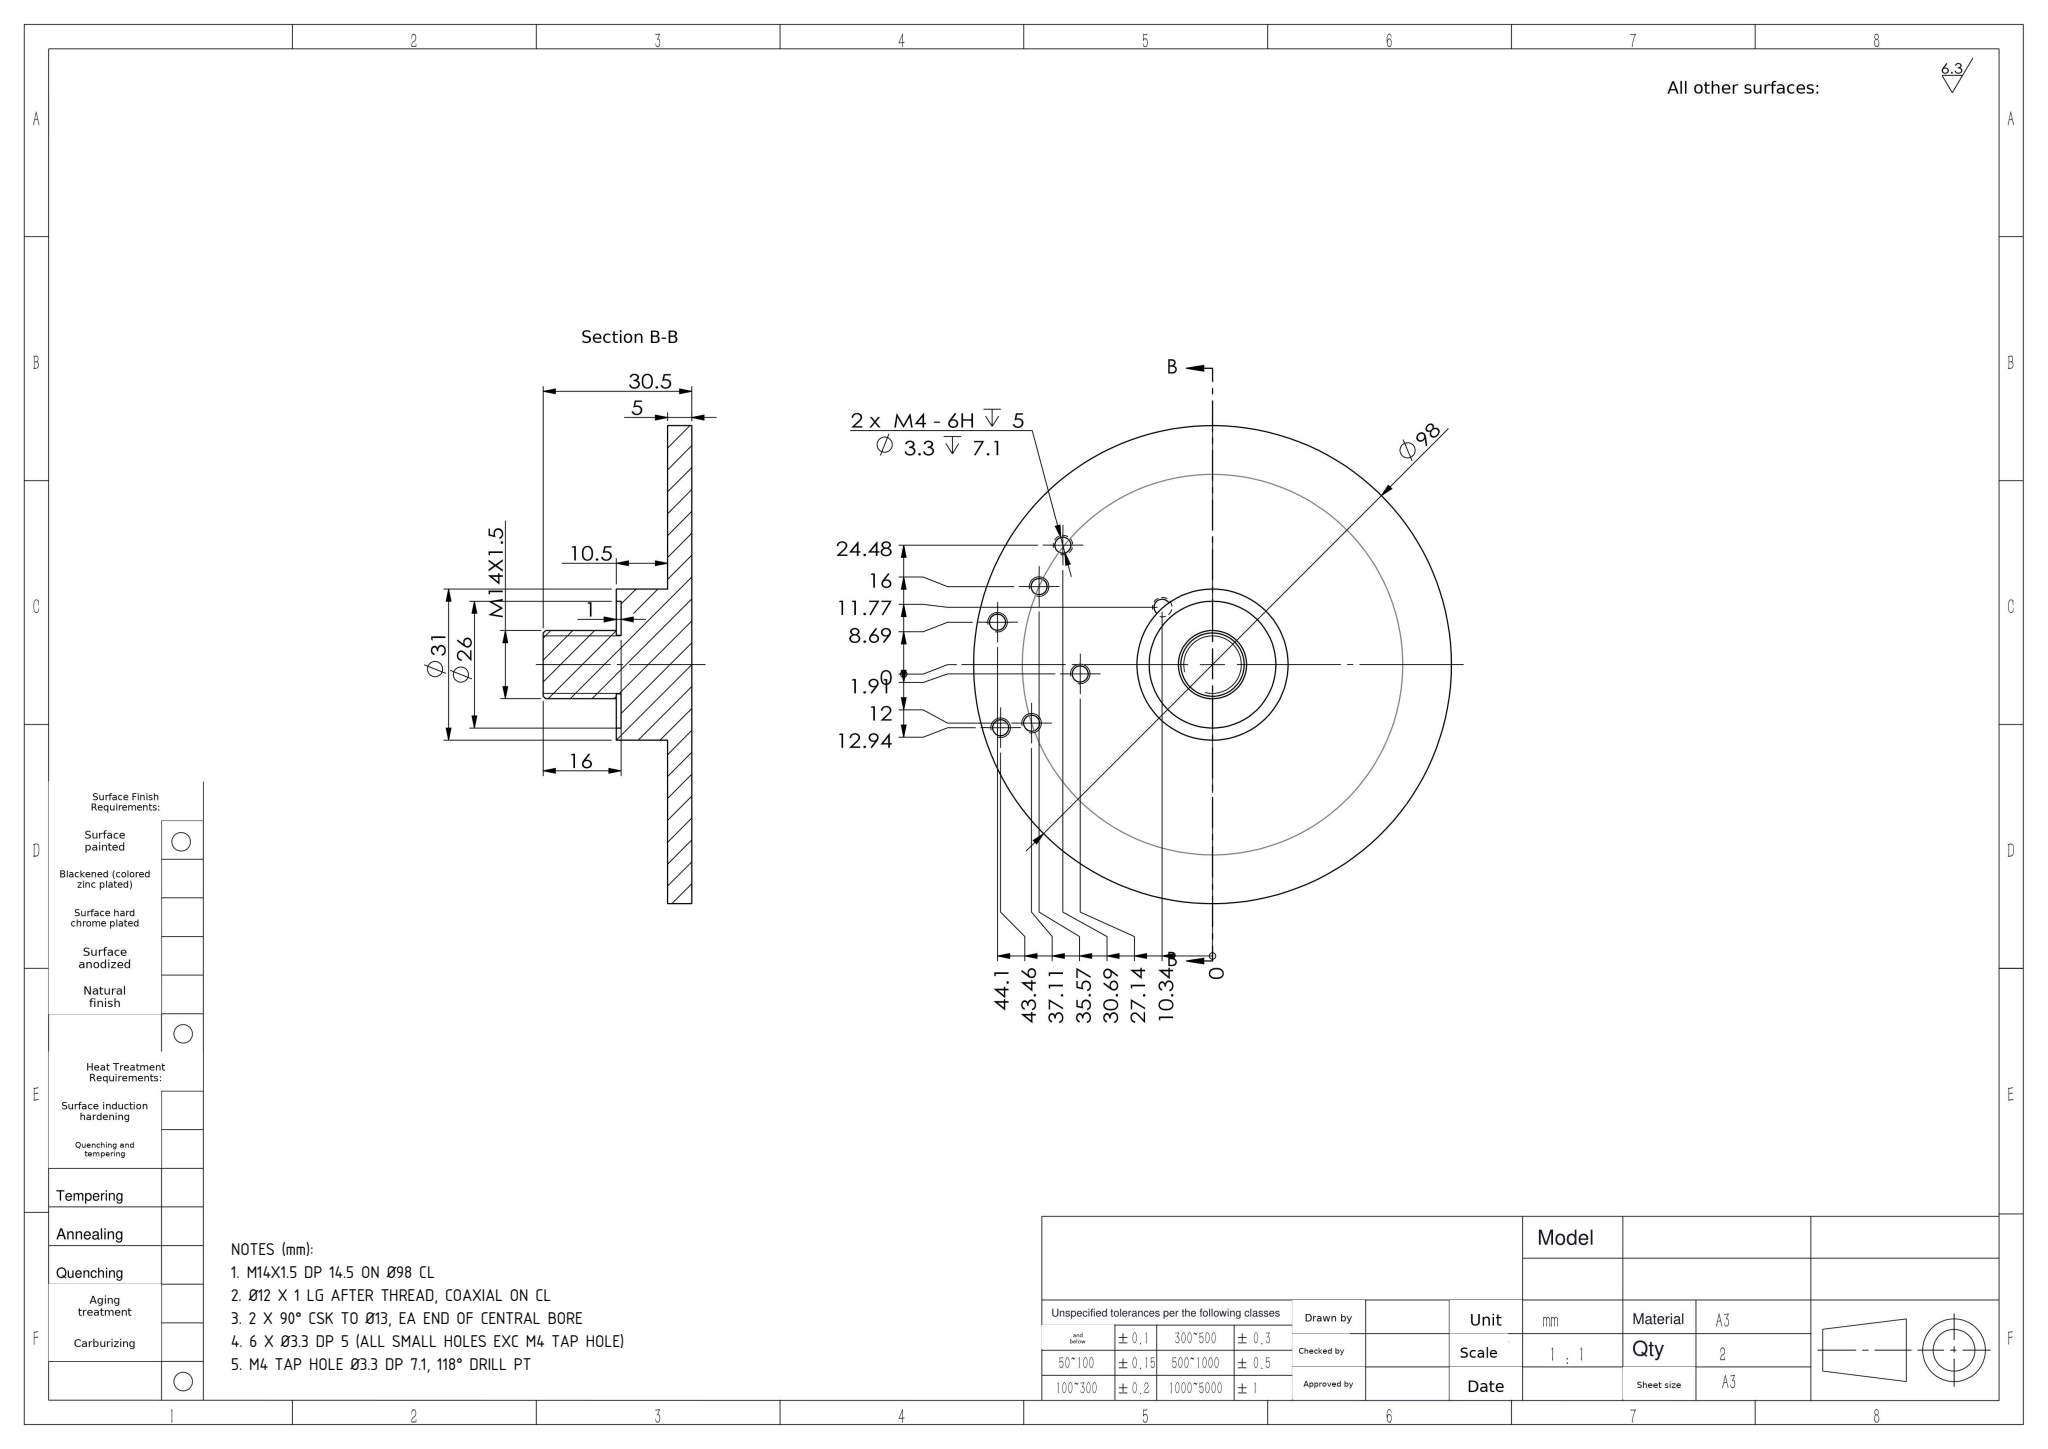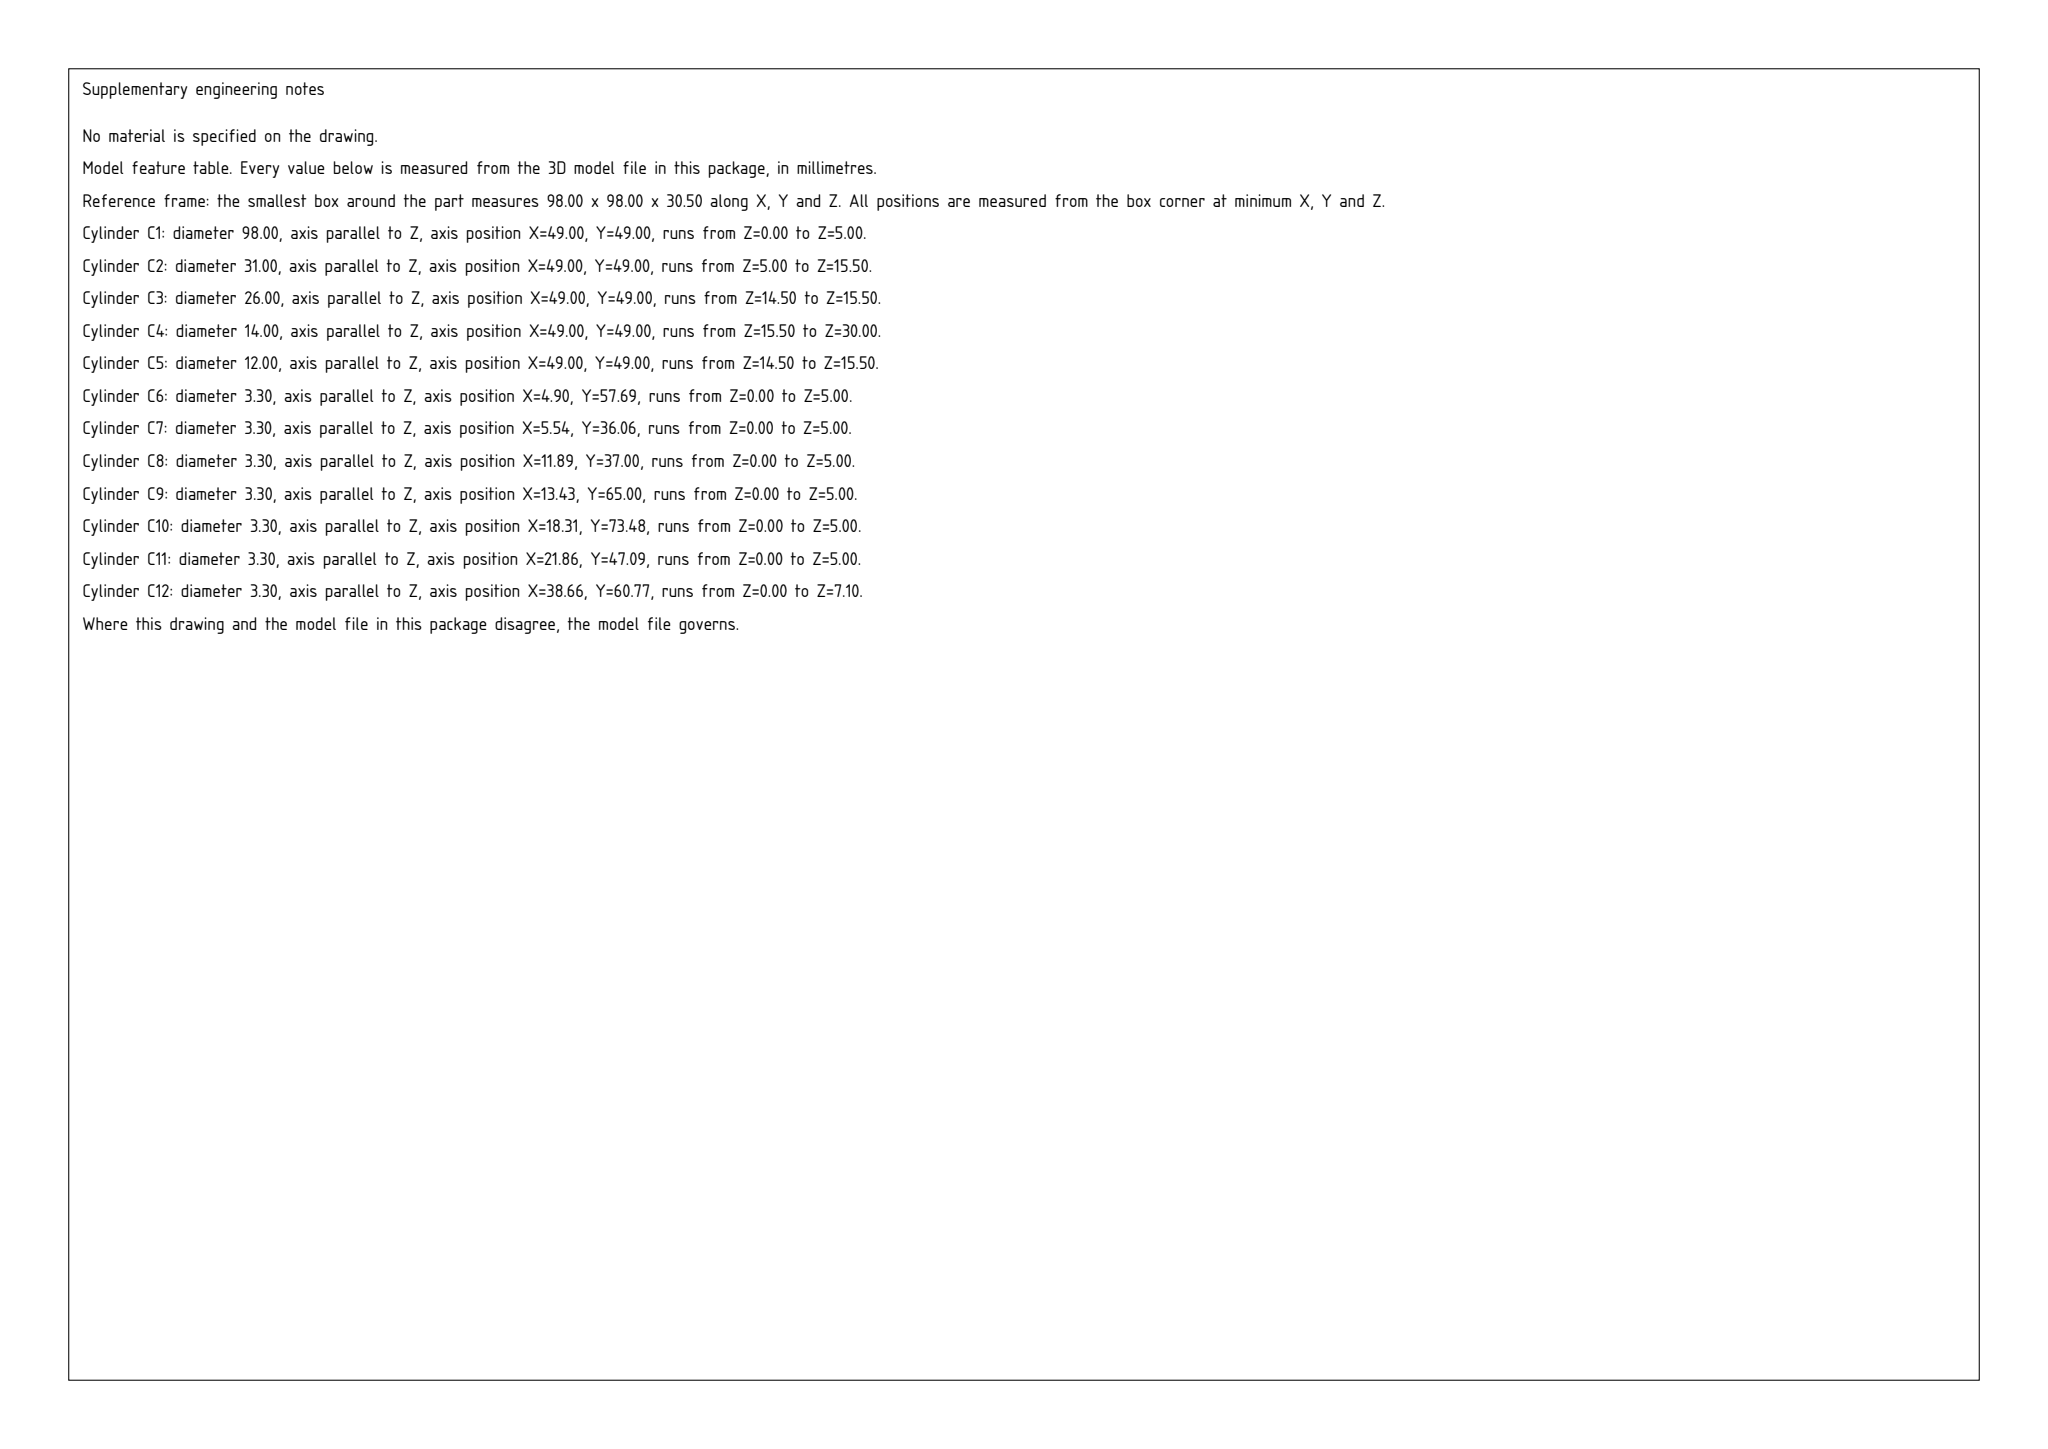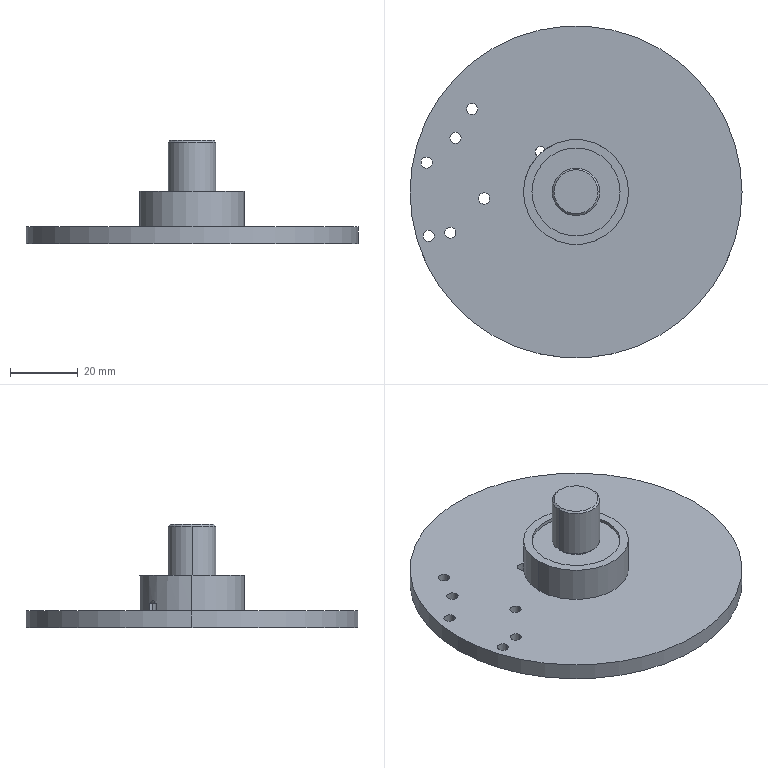Part | SolidWorks | mm | 1 solid | 33 faces | box 98 x 98 x 30.5 mm | volume 47218 mm3 | cylinder 24 | plane 6 | cone 3 | commonest cylinder face diameters 3.3 x14 14 x2 12 x2 26 x2 31 x2 98 x2
Drawing notes:
M14X1.5 DP 14.5 ON Ø98 CL | from the solid: cyl Ø14 axis z at (49,49) len 14.5; plane z=14.5
Ø12 X 1 LG AFTER THREAD, COAXIAL ON CL | from the solid: cyl Ø12 axis z at (49,49) len 1.0; planes z=14.5 and z=15.5
2 X 90° CSK TO Ø13, EA END OF CENTRAL BORE | from the solid: cones [90.0, ref dia 13.0, qty 2] coaxial with Ø12/Ø14 bore
6 X Ø3.3 DP 5 (ALL SMALL HOLES EXC M4 TAP HOLE) | from the solid: six cyl Ø3.3 axis z len 5.0 at (4.9,57.69),(5.54,36.06),(11.89,37.0),(13.43,65.0),(18.31,73.48),(21.86,47.09)
M4 TAP HOLE Ø3.3 DP 7.1, 118° DRILL PT | from the solid: cyl Ø3.3 len 7.1 at (38.66,60.77); cone 118° ref dia 3.3
build123d program:
from build123d import *

# Parameters (mm, degrees)
SKETCH1_R             = 49
BOSS_EXTRUDE1_DEPTH   = 5
SKETCH3_R             = 15.5
BOSS_EXTRUDE2_DEPTH   = 10.5
SKETCH4_R             = 7
BOSS_EXTRUDE3_DEPTH   = 15
M4_TAPPED_HOLE1_D     = 3.3
M4_TAPPED_HOLE3_D     = 3.3
M4_TAPPED_HOLE3_DEPTH = 7.1
M4_TAPPED_HOLE3_TIP   = 0.9914
M4_TAPPED_HOLE4_D     = 3.3
CUT_EXTRUDE1_START    = -1
SKETCH16_R            = 13
SKETCH16_R_2          = 7
CUT_EXTRUDE1_DEPTH    = 1
CHAMFER1_SIZE         = 0.5
SKETCH17_W            = 1
SKETCH17_H            = 1


with BuildPart() as part:
    # Sketch1 → Boss-Extrude1 (new body)
    with BuildSketch(Plane.XY):
        Circle(SKETCH1_R)
    extrude(amount=BOSS_EXTRUDE1_DEPTH)

    # Sketch3 → Boss-Extrude2 (add)
    with BuildSketch(Plane.XY.offset(5)):
        with Locations(Location((0, 0, 0), (0, 0, 180))):
            Circle(SKETCH3_R)
    extrude(amount=BOSS_EXTRUDE2_DEPTH)

    # Sketch4 → Boss-Extrude3 (add)
    with BuildSketch(Plane.XY.offset(15.5)):
        Circle(SKETCH4_R)
    extrude(amount=BOSS_EXTRUDE3_DEPTH)

    # M4 Tapped Hole1 (through all)
    with Locations(Plane.XY.offset(5)):
        with Locations((-35.567, 16), (-37.108, -12)):
            Hole(M4_TAPPED_HOLE1_D / 2)

    # M4 Tapped Hole3
    with Locations(Plane(origin=(0, 0, 0), x_dir=(-1, 0, 0), z_dir=(0, 0, -1))):
        with Locations((10.336, 11.765), (30.689, 24.483)):
            Hole(M4_TAPPED_HOLE3_D / 2, depth=M4_TAPPED_HOLE3_DEPTH)
            with Locations((0, 0, -(M4_TAPPED_HOLE3_DEPTH + M4_TAPPED_HOLE3_TIP / 2))):  # 118° drill point
                Cone(0, M4_TAPPED_HOLE3_D / 2, M4_TAPPED_HOLE3_TIP, mode=Mode.SUBTRACT)

    # M4 Tapped Hole4 (through all)
    with Locations(Plane(origin=(0, 0, 0), x_dir=(-1, 0, 0), z_dir=(0, 0, -1))):
        with Locations((27.136, -1.911), (44.097, 8.688), (43.459, -12.936)):
            Hole(M4_TAPPED_HOLE4_D / 2)

    # Sketch16 → Cut-Extrude1 (cut)
    with BuildSketch(Plane.XY.offset(15.5).offset(CUT_EXTRUDE1_START)):
        Circle(SKETCH16_R)
        Circle(SKETCH16_R_2, mode=Mode.SUBTRACT)
    extrude(amount=CUT_EXTRUDE1_DEPTH, mode=Mode.SUBTRACT)

    # Chamfer1
    chamfer1_edges = [part.edges().sort_by_distance(p)[0] for p in [
        (-7, 0, 30.5),
    ]]
    chamfer(chamfer1_edges, length=CHAMFER1_SIZE)

    # Sketch17 → Cut-Revolve1 (revolve, cut)
    with BuildSketch(Plane(origin=(0, 0, 0), x_dir=(0, 0, -1), z_dir=(1, 0, 0))):
        with Locations((-15, 6.5)):
            Rectangle(SKETCH17_W, SKETCH17_H)
    revolve(axis=Axis((0, 0, 0), (0, 0, 1)), mode=Mode.SUBTRACT)


solid = part.part